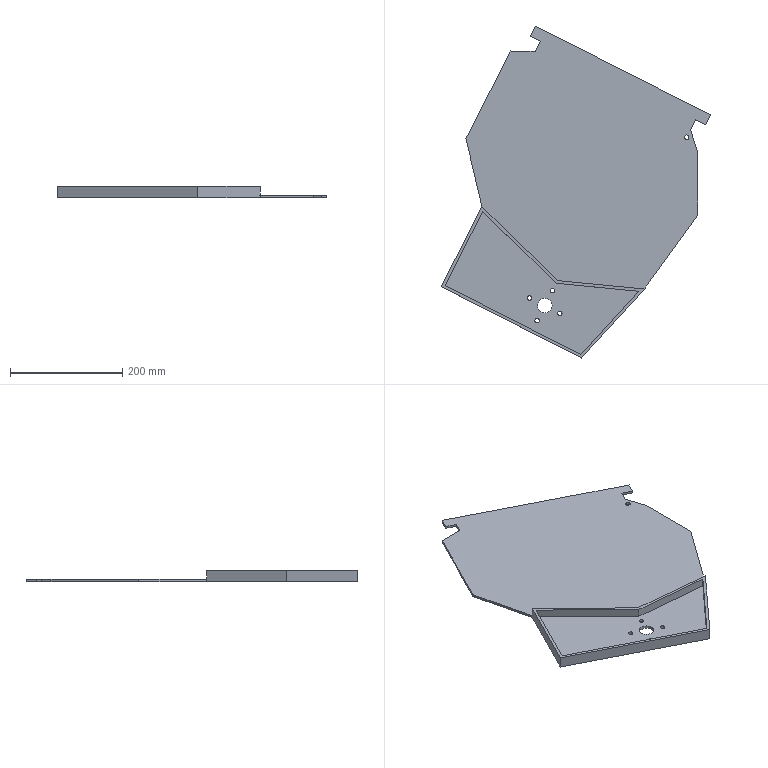Component | SolidWorks | SeedBoxAssemblyModified-1_SeedBoxLidModification-2 | 1 solid | 39 faces | volume 805757 mm3 | plane 27 | cylinder 12 | commonest cylinder face diameters 8 x10 26 x2